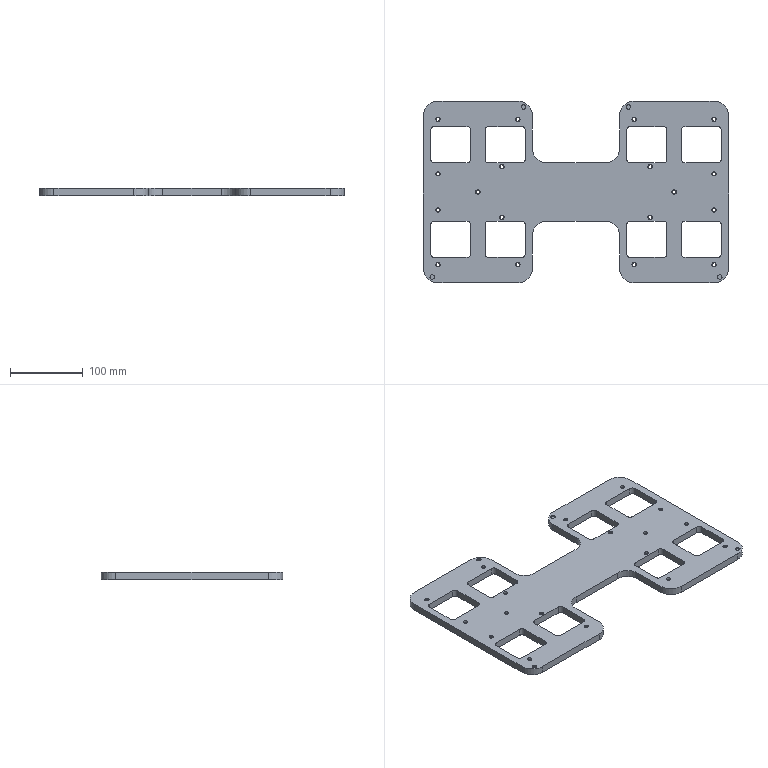Component | SolidWorks | Gripper-2024-3-4-04-1 | 1 solid | 195 faces | box 420 x 250 x 10 mm | volume 610506 mm3 | cylinder 126 | plane 69 | commonest cylinder face diameters 6 x44 5 x36 10 x32 40 x12 64 x2 | material AL6061
build123d program:
from build123d import *

# Parameters (mm, degrees)
SKETCH1_2_W                         = 420
SKETCH1_2_H                         = 270
BOSS_EXTRUDE1_DEPTH                 = 10
SKETCH2_2_W                         = 1000
SKETCH2_2_H                         = 10
CUT_EXTRUDE1_DEPTH                  = 500.4
SKETCH3_R                           = 3
CUT_EXTRUDE2_DEPTH                  = 2
M5_TAPPED_HOLE1_D                   = 5
SKETCH6_W                           = 120
SKETCH6_H                           = 85
CUT_EXTRUDE3_DEPTH                  = 495.065
FILLET1_R                           = 20
CUT_EXTRUDE4_DEPTH                  = 495.065
SKETCH8_R                           = 32
CUT_EXTRUDE5_DEPTH                  = 3
SKETCH1_R                           = 3
RODSEAT_R_MIRROR_OF_CUT2_DEPTH      = 2
SKETCH2_R                           = 3
PINTHREADRUNOUTRELIEF_D6X2_35_DEPTH = 2.35


with BuildPart() as part:
    # Sketch1_2 → Boss-Extrude1 (new body)
    with BuildSketch(Plane.XY):
        with Locations((210, 135)):
            Rectangle(SKETCH1_2_W, SKETCH1_2_H)
    extrude(amount=BOSS_EXTRUDE1_DEPTH)

    # Sketch2_2 → Cut-Extrude1 (cut, through all)
    with BuildSketch(Plane.XY.offset(10)):
        with Locations((500, 265)):
            Rectangle(SKETCH2_2_W, SKETCH2_2_H)
        with Locations((500, 5)):
            Rectangle(SKETCH2_2_W, SKETCH2_2_H)
    extrude(amount=-CUT_EXTRUDE1_DEPTH, mode=Mode.SUBTRACT)

    # Sketch3 → Cut-Extrude2 (cut)
    with BuildSketch(Plane.XY.offset(10)):
        with Locations((12, 18)):
            Circle(SKETCH3_R)
        with Locations((138, 252)):
            Circle(SKETCH3_R)
    extrude(amount=-CUT_EXTRUDE2_DEPTH, mode=Mode.SUBTRACT)

    # M5 Tapped Hole1 (through all)
    with Locations(Plane.XY.offset(10)):
        with Locations((20, 35), (130, 35), (75, 135), (108, 100), (20, 110), (20, 160), (108, 170), (130, 235), (20, 235), (400, 235), (290, 235), (312, 170), (400, 160), (400, 110), (312, 100), (345, 135), (290, 35), (400, 35)):
            Hole(M5_TAPPED_HOLE1_D / 2)

    # Sketch6 → Cut-Extrude3 (cut, through all)
    with BuildSketch(Plane.XY.offset(10)):
        with Locations((210, 217.5)):
            Rectangle(SKETCH6_W, SKETCH6_H)
        with Locations((210, 52.5)):
            Rectangle(SKETCH6_W, SKETCH6_H)
    extrude(amount=-CUT_EXTRUDE3_DEPTH, mode=Mode.SUBTRACT)

    # Fillet1
    fillet1_edges = [part.edges().sort_by_distance(p)[0] for p in [
        (420, 260, 5),
        (150, 10, 5),
        (150, 95, 5),
        (270, 95, 5),
        (270, 10, 5),
        (270, 260, 5),
        (270, 175, 5),
        (150, 175, 5),
        (150, 260, 5),
        (0, 260, 5),
        (420, 10, 5),
        (0, 10, 5),
    ]]
    fillet(fillet1_edges, radius=FILLET1_R)

    # Sketch7 → Cut-Extrude4 (cut, through all)
    with BuildSketch(Plane(origin=(0, 0, 0), x_dir=(-1, 0, 0), z_dir=(0, 0, -1))):
        with BuildLine():
            Line((-405, 225), (-360, 225))
            ThreePointArc((-360, 225), (-356.464, 223.536), (-355, 220))
            Line((-355, 220), (-355, 180))
            ThreePointArc((-355, 180), (-356.464, 176.464), (-360, 175))
            Line((-360, 175), (-405, 175))
            ThreePointArc((-405, 175), (-408.536, 176.464), (-410, 180))
            Line((-410, 180), (-410, 220))
            ThreePointArc((-410, 220), (-408.536, 223.536), (-405, 225))
        make_face()
        with BuildLine():
            Line((-285, 175), (-330, 175))
            ThreePointArc((-330, 175), (-333.536, 176.464), (-335, 180))
            Line((-335, 180), (-335, 220))
            ThreePointArc((-335, 220), (-333.536, 223.536), (-330, 225))
            Line((-330, 225), (-285, 225))
            ThreePointArc((-285, 225), (-281.464, 223.536), (-280, 220))
            Line((-280, 220), (-280, 180))
            ThreePointArc((-280, 180), (-281.464, 176.464), (-285, 175))
        make_face()
        with BuildLine():
            Line((-280, 50), (-280, 90))
            ThreePointArc((-280, 90), (-281.464, 93.536), (-285, 95))
            Line((-285, 95), (-330, 95))
            ThreePointArc((-330, 95), (-333.536, 93.536), (-335, 90))
            Line((-335, 90), (-335, 50))
            ThreePointArc((-335, 50), (-333.536, 46.464), (-330, 45))
            Line((-330, 45), (-285, 45))
            ThreePointArc((-285, 45), (-281.464, 46.464), (-280, 50))
        make_face()
        with BuildLine():
            Line((-405, 95), (-360, 95))
            ThreePointArc((-360, 95), (-356.464, 93.536), (-355, 90))
            Line((-355, 90), (-355, 50))
            ThreePointArc((-355, 50), (-356.464, 46.464), (-360, 45))
            Line((-360, 45), (-405, 45))
            ThreePointArc((-405, 45), (-408.536, 46.464), (-410, 50))
            Line((-410, 50), (-410, 90))
            ThreePointArc((-410, 90), (-408.536, 93.536), (-405, 95))
        make_face()
        with BuildLine():
            Line((-10, 50), (-10, 90))
            ThreePointArc((-10, 90), (-11.464, 93.536), (-15, 95))
            Line((-15, 95), (-60, 95))
            ThreePointArc((-60, 95), (-63.536, 93.536), (-65, 90))
            Line((-65, 90), (-65, 50))
            ThreePointArc((-65, 50), (-63.536, 46.464), (-60, 45))
            Line((-60, 45), (-15, 45))
            ThreePointArc((-15, 45), (-11.464, 46.464), (-10, 50))
        make_face()
        with BuildLine():
            Line((-135, 95), (-90, 95))
            ThreePointArc((-90, 95), (-86.464, 93.536), (-85, 90))
            Line((-85, 90), (-85, 50))
            ThreePointArc((-85, 50), (-86.464, 46.464), (-90, 45))
            Line((-90, 45), (-135, 45))
            ThreePointArc((-135, 45), (-138.536, 46.464), (-140, 50))
            Line((-140, 50), (-140, 90))
            ThreePointArc((-140, 90), (-138.536, 93.536), (-135, 95))
        make_face()
        with BuildLine():
            Line((-140, 220), (-140, 180))
            ThreePointArc((-140, 180), (-138.536, 176.464), (-135, 175))
            Line((-135, 175), (-90, 175))
            ThreePointArc((-90, 175), (-86.464, 176.464), (-85, 180))
            Line((-85, 180), (-85, 220))
            ThreePointArc((-85, 220), (-86.464, 223.536), (-90, 225))
            Line((-90, 225), (-135, 225))
            ThreePointArc((-135, 225), (-138.536, 223.536), (-140, 220))
        make_face()
        with BuildLine():
            Line((-65, 220), (-65, 180))
            ThreePointArc((-65, 180), (-63.536, 176.464), (-60, 175))
            Line((-60, 175), (-15, 175))
            ThreePointArc((-15, 175), (-11.464, 176.464), (-10, 180))
            Line((-10, 180), (-10, 220))
            ThreePointArc((-10, 220), (-11.464, 223.536), (-15, 225))
            Line((-15, 225), (-60, 225))
            ThreePointArc((-60, 225), (-63.536, 223.536), (-65, 220))
        make_face()
    extrude(amount=-CUT_EXTRUDE4_DEPTH, mode=Mode.SUBTRACT)

    # Sketch8 → Cut-Extrude5 (cut)
    with BuildSketch(Plane(origin=(0, 0, 0), x_dir=(-1, 0, 0), z_dir=(0, 0, -1))):
        with Locations((-210, 135)):
            Circle(SKETCH8_R)
    extrude(amount=-CUT_EXTRUDE5_DEPTH, mode=Mode.SUBTRACT)

    # Sketch1 → RodSeat_R_mirror_of_Cut2 (cut)
    with BuildSketch(Plane.XY.offset(10)):
        with Locations((282, 252)):
            Circle(SKETCH1_R)
        with Locations((408, 18)):
            Circle(SKETCH1_R)
    extrude(amount=-RODSEAT_R_MIRROR_OF_CUT2_DEPTH, mode=Mode.SUBTRACT)

    # Sketch2 → PinThreadRunoutRelief_D6x2_35 (cut)
    with BuildSketch(Plane.XY.offset(10)):
        with Locations((20, 235)):
            Circle(SKETCH2_R)
        with Locations((130, 235)):
            Circle(SKETCH2_R)
        with Locations((108, 170)):
            Circle(SKETCH2_R)
        with Locations((400, 160)):
            Circle(SKETCH2_R)
        with Locations((20, 160)):
            Circle(SKETCH2_R)
        with Locations((290, 35)):
            Circle(SKETCH2_R)
        with Locations((400, 235)):
            Circle(SKETCH2_R)
        with Locations((312, 170)):
            Circle(SKETCH2_R)
        with Locations((400, 35)):
            Circle(SKETCH2_R)
        with Locations((290, 235)):
            Circle(SKETCH2_R)
        with Locations((345, 135)):
            Circle(SKETCH2_R)
        with Locations((400, 110)):
            Circle(SKETCH2_R)
        with Locations((312, 100)):
            Circle(SKETCH2_R)
        with Locations((108, 100)):
            Circle(SKETCH2_R)
        with Locations((75, 135)):
            Circle(SKETCH2_R)
        with Locations((20, 110)):
            Circle(SKETCH2_R)
        with Locations((20, 35)):
            Circle(SKETCH2_R)
        with Locations((130, 35)):
            Circle(SKETCH2_R)
    extrude(amount=-PINTHREADRUNOUTRELIEF_D6X2_35_DEPTH, mode=Mode.SUBTRACT)


solid = part.part

# Placed as in the assembly
solid = solid.moved(Location((-175.094, -141.769, 295), (0, 0, 0)))